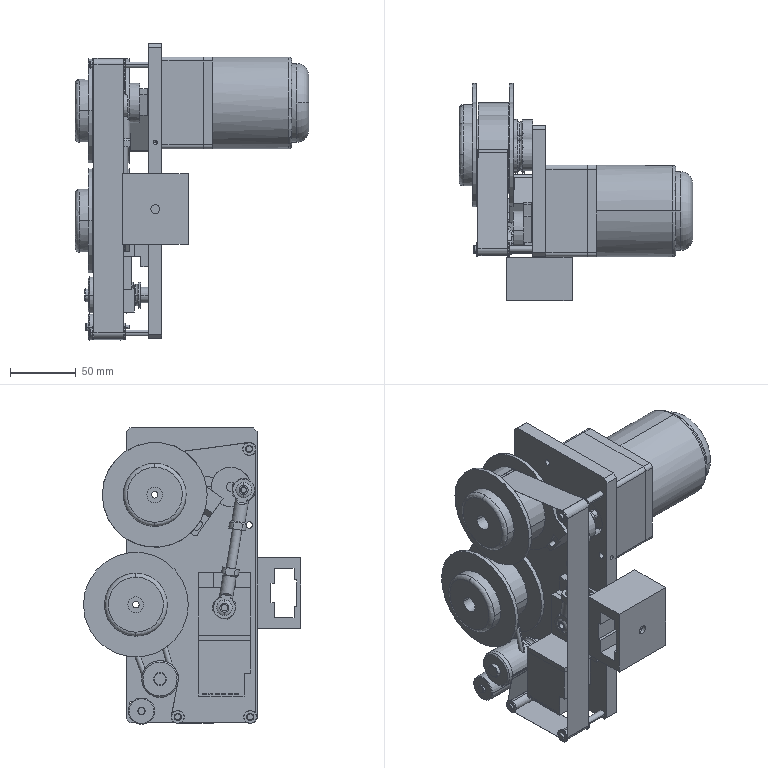Component | SolidWorks | FilmMechanism-3-1_CodingMachine-1 | 17 solids | 640 faces | volume 1069024 mm3 | cylinder 263 | plane 259 | torus 78 | cone 36 | sphere 4 | commonest cylinder face diameters 0.4 x36 6 x32 5 x28 10 x23 4 x16 25 x16 8 x12 12 x10